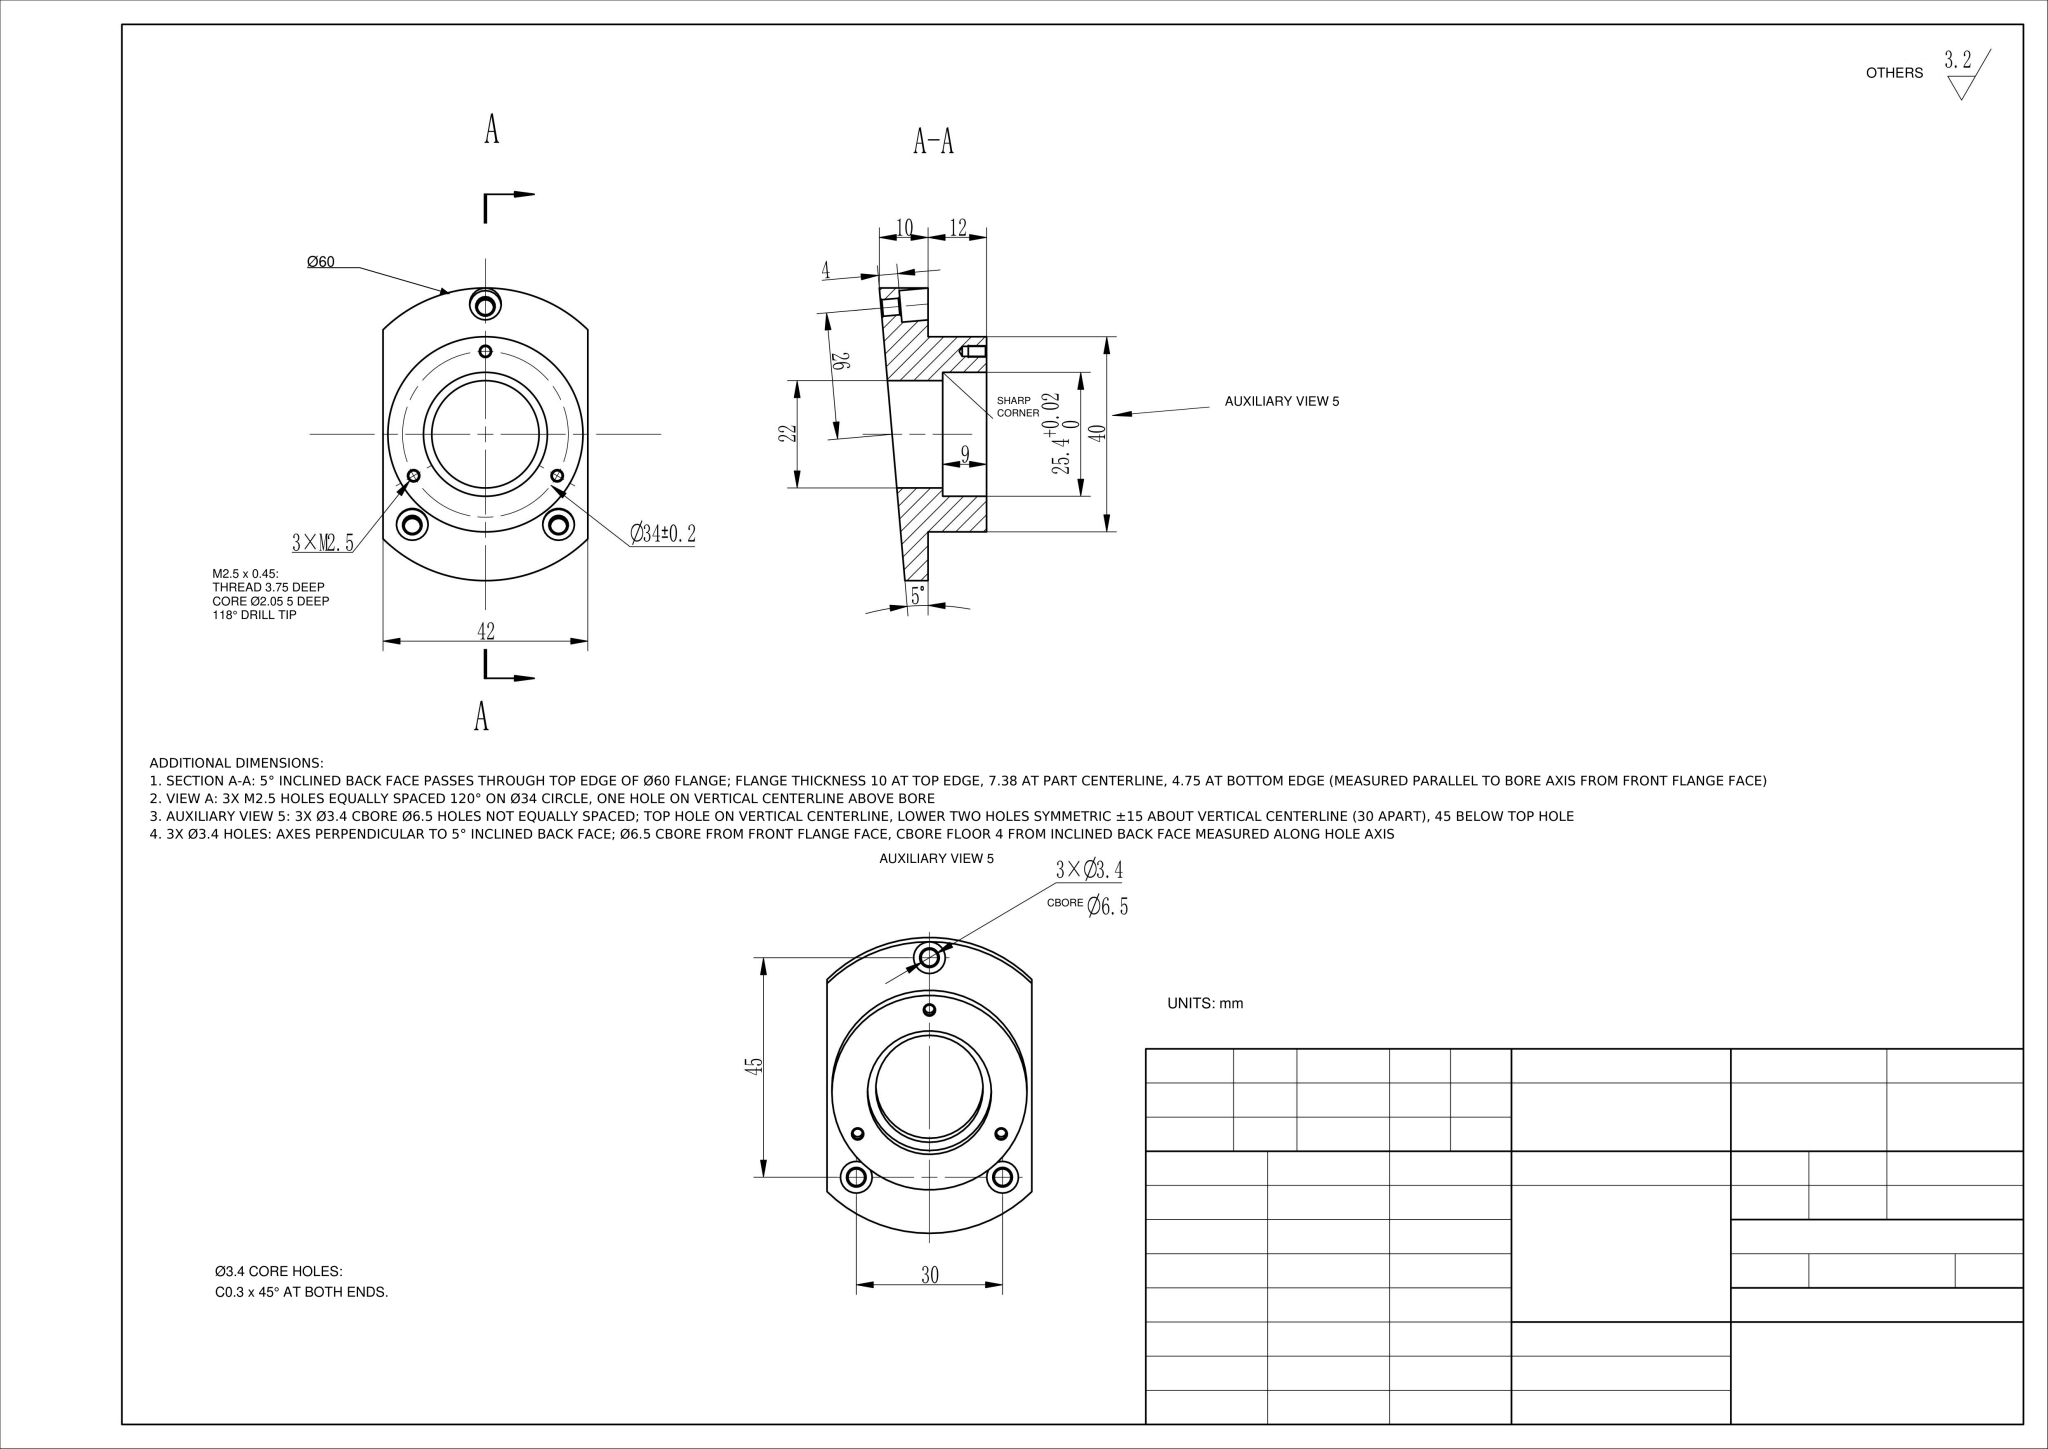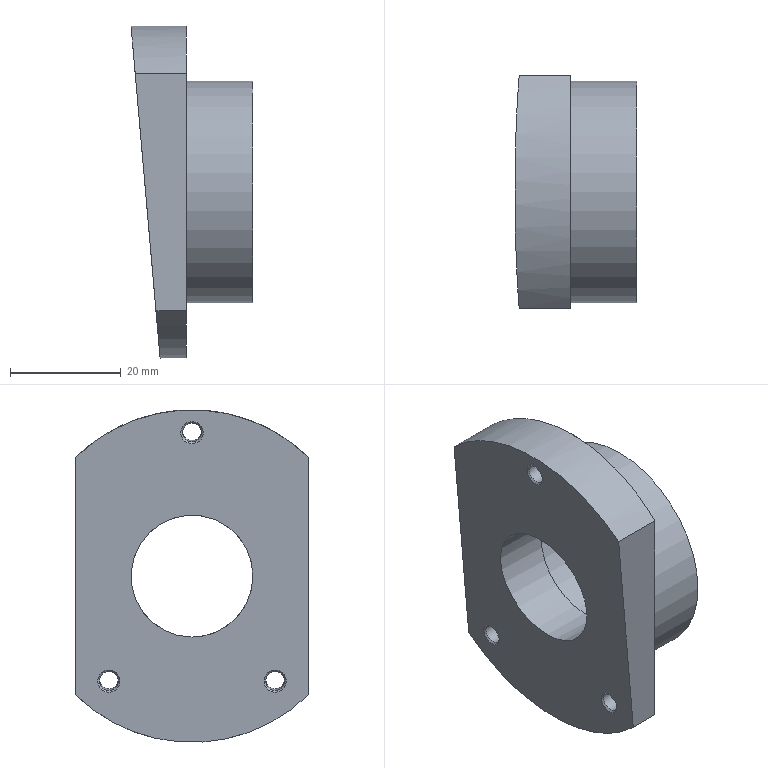Part | NX | mm | 1 solid | 35 faces | box 22 x 42 x 60 mm | volume 23038 mm3 | cylinder 14 | cone 12 | plane 9 | commonest cylinder face diameters 2.05 x3 6.5 x3 3.4 x3 60 x2 22 x1 40 x1 25.4 x1
STEP:
#1=CARTESIAN_POINT('',(0.,0.,0.));
#2=DIRECTION('',(0.,0.,1.));
#3=DIRECTION('',(1.,0.,0.));
#4=AXIS2_PLACEMENT_3D('',#1,#2,#3);
#5=(LENGTH_UNIT()NAMED_UNIT(*)SI_UNIT(.MILLI.,.METRE.));
#6=UNCERTAINTY_MEASURE_WITH_UNIT(LENGTH_MEASURE(0.00002),#5,'','');
#7=(NAMED_UNIT(*)PLANE_ANGLE_UNIT()SI_UNIT($,.RADIAN.));
#8=PLANE_ANGLE_MEASURE_WITH_UNIT(PLANE_ANGLE_MEASURE(0.01745),#7);
#9=DIMENSIONAL_EXPONENTS(0.,0.,0.,0.,0.,0.,0.);
#10=(CONVERSION_BASED_UNIT('',#8)NAMED_UNIT(#9)PLANE_ANGLE_UNIT());
#11=(NAMED_UNIT(*)SI_UNIT($,.STERADIAN.)SOLID_ANGLE_UNIT());
#12=(GEOMETRIC_REPRESENTATION_CONTEXT(3)GLOBAL_UNCERTAINTY_ASSIGNED_CONTEXT((#6))GLOBAL_UNIT_ASSIGNED_CONTEXT((#5,#10,#11))REPRESENTATION_CONTEXT('',''));
#13=SHAPE_REPRESENTATION('',(#4),#12);
#14=CARTESIAN_POINT('',(-5.501,-21.,-21.424));
#15=VERTEX_POINT('',#14);
#16=CARTESIAN_POINT('',(-9.25,-21.,21.424));
#17=VERTEX_POINT('',#16);
#18=CARTESIAN_POINT('',(-4.751,-21.,-30.));
#19=DIRECTION('',(-0.08716,0.,0.9962));
#20=VECTOR('',#19,1.);
#21=LINE('',#18,#20);
#22=EDGE_CURVE('',#15,#17,#21,.T.);
#23=ORIENTED_EDGE('',*,*,#22,.F.);
#24=CARTESIAN_POINT('',(0.,-21.,-21.424));
#25=VERTEX_POINT('',#24);
#26=CARTESIAN_POINT('',(-10.,-21.,-21.424));
#27=DIRECTION('',(1.,0.,0.));
#28=VECTOR('',#27,1.);
#29=LINE('',#26,#28);
#30=EDGE_CURVE('',#15,#25,#29,.T.);
#31=ORIENTED_EDGE('',*,*,#30,.T.);
#32=CARTESIAN_POINT('',(0.,-21.,21.424));
#33=VERTEX_POINT('',#32);
#34=CARTESIAN_POINT('',(0.,-21.,-21.424));
#35=DIRECTION('',(0.,-0.,1.));
#36=VECTOR('',#35,1.);
#37=LINE('',#34,#36);
#38=EDGE_CURVE('',#25,#33,#37,.T.);
#39=ORIENTED_EDGE('',*,*,#38,.T.);
#40=CARTESIAN_POINT('',(-10.,-21.,21.424));
#41=DIRECTION('',(1.,0.,0.));
#42=VECTOR('',#41,1.);
#43=LINE('',#40,#42);
#44=EDGE_CURVE('',#17,#33,#43,.T.);
#45=ORIENTED_EDGE('',*,*,#44,.F.);
#46=EDGE_LOOP('',(#23,#31,#39,#45));
#47=FACE_OUTER_BOUND('',#46,.T.);
#48=CARTESIAN_POINT('',(-10.,-21.,-21.424));
#49=DIRECTION('',(0.,1.,0.));
#50=DIRECTION('',(0.,-0.,1.));
#51=AXIS2_PLACEMENT_3D('',#48,#49,#50);
#52=PLANE('',#51);
#53=ADVANCED_FACE('',(#47),#52,.F.);
#54=CARTESIAN_POINT('',(3.,0.,-11.));
#55=VERTEX_POINT('',#54);
#56=CARTESIAN_POINT('',(3.,0.,0.));
#57=DIRECTION('',(-1.,0.,0.));
#58=DIRECTION('',(0.,0.,-1.));
#59=AXIS2_PLACEMENT_3D('',#56,#57,#58);
#60=CIRCLE('',#59,11.);
#61=EDGE_CURVE('',#55,#55,#60,.T.);
#62=ORIENTED_EDGE('',*,*,#61,.F.);
#63=EDGE_LOOP('',(#62));
#64=FACE_BOUND('',#63,.T.);
#65=CARTESIAN_POINT('',(-6.413,0.,-11.));
#66=VERTEX_POINT('',#65);
#67=CARTESIAN_POINT('',(-7.375,0.,0.));
#68=DIRECTION('',(0.9962,0.,0.08716));
#69=DIRECTION('',(0.08716,0.,-0.9962));
#70=AXIS2_PLACEMENT_3D('',#67,#68,#69);
#71=ELLIPSE('',#70,11.042,11.);
#72=EDGE_CURVE('',#66,#66,#71,.T.);
#73=ORIENTED_EDGE('',*,*,#72,.F.);
#74=EDGE_LOOP('',(#73));
#75=FACE_BOUND('',#74,.T.);
#76=CARTESIAN_POINT('',(-4.,0.,0.));
#77=DIRECTION('',(1.,0.,0.));
#78=DIRECTION('',(0.,0.,-1.));
#79=AXIS2_PLACEMENT_3D('',#76,#77,#78);
#80=CYLINDRICAL_SURFACE('',#79,11.);
#81=ADVANCED_FACE('',(#64,#75),#80,.F.);
#82=CARTESIAN_POINT('',(-9.25,21.,21.424));
#83=VERTEX_POINT('',#82);
#84=CARTESIAN_POINT('',(-7.375,0.,0.));
#85=DIRECTION('',(-0.9962,0.,-0.08716));
#86=DIRECTION('',(0.08716,0.,-0.9962));
#87=AXIS2_PLACEMENT_3D('',#84,#85,#86);
#88=ELLIPSE('',#87,30.115,30.);
#89=EDGE_CURVE('',#17,#83,#88,.T.);
#90=ORIENTED_EDGE('',*,*,#89,.F.);
#91=ORIENTED_EDGE('',*,*,#44,.T.);
#92=CARTESIAN_POINT('',(0.,21.,21.424));
#93=VERTEX_POINT('',#92);
#94=CARTESIAN_POINT('',(0.,0.,0.));
#95=DIRECTION('',(-1.,0.,0.));
#96=DIRECTION('',(0.,-1.,-0.));
#97=AXIS2_PLACEMENT_3D('',#94,#95,#96);
#98=CIRCLE('',#97,30.);
#99=EDGE_CURVE('',#33,#93,#98,.T.);
#100=ORIENTED_EDGE('',*,*,#99,.T.);
#101=CARTESIAN_POINT('',(-10.,21.,21.424));
#102=DIRECTION('',(1.,0.,0.));
#103=VECTOR('',#102,1.);
#104=LINE('',#101,#103);
#105=EDGE_CURVE('',#83,#93,#104,.T.);
#106=ORIENTED_EDGE('',*,*,#105,.F.);
#107=EDGE_LOOP('',(#90,#91,#100,#106));
#108=FACE_OUTER_BOUND('',#107,.T.);
#109=CARTESIAN_POINT('',(-10.,0.,0.));
#110=DIRECTION('',(1.,0.,0.));
#111=DIRECTION('',(0.,0.,-1.));
#112=AXIS2_PLACEMENT_3D('',#109,#110,#111);
#113=CYLINDRICAL_SURFACE('',#112,30.);
#114=ADVANCED_FACE('',(#108),#113,.T.);
#115=ORIENTED_EDGE('',*,*,#30,.F.);
#116=CARTESIAN_POINT('',(-5.501,21.,-21.424));
#117=VERTEX_POINT('',#116);
#118=CARTESIAN_POINT('',(-7.375,0.,0.));
#119=DIRECTION('',(-0.9962,0.,-0.08716));
#120=DIRECTION('',(0.08716,0.,-0.9962));
#121=AXIS2_PLACEMENT_3D('',#118,#119,#120);
#122=ELLIPSE('',#121,30.115,30.);
#123=EDGE_CURVE('',#117,#15,#122,.T.);
#124=ORIENTED_EDGE('',*,*,#123,.F.);
#125=CARTESIAN_POINT('',(0.,21.,-21.424));
#126=VERTEX_POINT('',#125);
#127=CARTESIAN_POINT('',(-10.,21.,-21.424));
#128=DIRECTION('',(1.,0.,0.));
#129=VECTOR('',#128,1.);
#130=LINE('',#127,#129);
#131=EDGE_CURVE('',#117,#126,#130,.T.);
#132=ORIENTED_EDGE('',*,*,#131,.T.);
#133=CARTESIAN_POINT('',(0.,0.,0.));
#134=DIRECTION('',(-1.,0.,0.));
#135=DIRECTION('',(0.,-1.,-0.));
#136=AXIS2_PLACEMENT_3D('',#133,#134,#135);
#137=CIRCLE('',#136,30.);
#138=EDGE_CURVE('',#126,#25,#137,.T.);
#139=ORIENTED_EDGE('',*,*,#138,.T.);
#140=EDGE_LOOP('',(#115,#124,#132,#139));
#141=FACE_OUTER_BOUND('',#140,.T.);
#142=CARTESIAN_POINT('',(-10.,0.,0.));
#143=DIRECTION('',(1.,0.,0.));
#144=DIRECTION('',(0.,0.,-1.));
#145=AXIS2_PLACEMENT_3D('',#142,#143,#144);
#146=CYLINDRICAL_SURFACE('',#145,30.);
#147=ADVANCED_FACE('',(#141),#146,.T.);
#148=CARTESIAN_POINT('',(12.,20.,-0.));
#149=VERTEX_POINT('',#148);
#150=CARTESIAN_POINT('',(12.,0.,0.));
#151=DIRECTION('',(1.,0.,0.));
#152=DIRECTION('',(0.,1.,-0.));
#153=AXIS2_PLACEMENT_3D('',#150,#151,#152);
#154=CIRCLE('',#153,20.);
#155=EDGE_CURVE('',#149,#149,#154,.T.);
#156=ORIENTED_EDGE('',*,*,#155,.F.);
#157=EDGE_LOOP('',(#156));
#158=FACE_BOUND('',#157,.T.);
#159=CARTESIAN_POINT('',(0.,20.,-0.));
#160=VERTEX_POINT('',#159);
#161=CARTESIAN_POINT('',(0.,0.,0.));
#162=DIRECTION('',(1.,0.,0.));
#163=DIRECTION('',(0.,1.,-0.));
#164=AXIS2_PLACEMENT_3D('',#161,#162,#163);
#165=CIRCLE('',#164,20.);
#166=EDGE_CURVE('',#160,#160,#165,.T.);
#167=ORIENTED_EDGE('',*,*,#166,.T.);
#168=EDGE_LOOP('',(#167));
#169=FACE_BOUND('',#168,.T.);
#170=CARTESIAN_POINT('',(12.,0.,0.));
#171=DIRECTION('',(-1.,0.,0.));
#172=DIRECTION('',(0.,0.,1.));
#173=AXIS2_PLACEMENT_3D('',#170,#171,#172);
#174=CYLINDRICAL_SURFACE('',#173,20.);
#175=ADVANCED_FACE('',(#158,#169),#174,.T.);
#176=CARTESIAN_POINT('',(12.,14.722,-9.75));
#177=VERTEX_POINT('',#176);
#178=CARTESIAN_POINT('',(12.,14.722,-8.5));
#179=DIRECTION('',(-1.,0.,0.));
#180=DIRECTION('',(0.,0.,-1.));
#181=AXIS2_PLACEMENT_3D('',#178,#179,#180);
#182=CIRCLE('',#181,1.25);
#183=EDGE_CURVE('',#177,#177,#182,.T.);
#184=ORIENTED_EDGE('',*,*,#183,.T.);
#185=EDGE_LOOP('',(#184));
#186=FACE_BOUND('',#185,.T.);
#187=CARTESIAN_POINT('',(12.,0.,15.75));
#188=VERTEX_POINT('',#187);
#189=CARTESIAN_POINT('',(12.,0.,17.));
#190=DIRECTION('',(-1.,0.,0.));
#191=DIRECTION('',(0.,0.,-1.));
#192=AXIS2_PLACEMENT_3D('',#189,#190,#191);
#193=CIRCLE('',#192,1.25);
#194=EDGE_CURVE('',#188,#188,#193,.T.);
#195=ORIENTED_EDGE('',*,*,#194,.T.);
#196=EDGE_LOOP('',(#195));
#197=FACE_BOUND('',#196,.T.);
#198=CARTESIAN_POINT('',(12.,-14.722,-9.75));
#199=VERTEX_POINT('',#198);
#200=CARTESIAN_POINT('',(12.,-14.722,-8.5));
#201=DIRECTION('',(-1.,0.,0.));
#202=DIRECTION('',(0.,0.,-1.));
#203=AXIS2_PLACEMENT_3D('',#200,#201,#202);
#204=CIRCLE('',#203,1.25);
#205=EDGE_CURVE('',#199,#199,#204,.T.);
#206=ORIENTED_EDGE('',*,*,#205,.T.);
#207=EDGE_LOOP('',(#206));
#208=FACE_BOUND('',#207,.T.);
#209=CARTESIAN_POINT('',(12.,12.7,-0.));
#210=VERTEX_POINT('',#209);
#211=CARTESIAN_POINT('',(12.,0.,0.));
#212=DIRECTION('',(1.,0.,0.));
#213=DIRECTION('',(0.,1.,-0.));
#214=AXIS2_PLACEMENT_3D('',#211,#212,#213);
#215=CIRCLE('',#214,12.7);
#216=EDGE_CURVE('',#210,#210,#215,.T.);
#217=ORIENTED_EDGE('',*,*,#216,.F.);
#218=EDGE_LOOP('',(#217));
#219=FACE_BOUND('',#218,.T.);
#220=ORIENTED_EDGE('',*,*,#155,.T.);
#221=EDGE_LOOP('',(#220));
#222=FACE_BOUND('',#221,.T.);
#223=CARTESIAN_POINT('',(12.,0.,0.));
#224=DIRECTION('',(1.,0.,0.));
#225=DIRECTION('',(0.,0.,-1.));
#226=AXIS2_PLACEMENT_3D('',#223,#224,#225);
#227=PLANE('',#226);
#228=ADVANCED_FACE('',(#186,#197,#208,#219,#222),#227,.T.);
#229=CARTESIAN_POINT('',(3.,12.7,-0.));
#230=VERTEX_POINT('',#229);
#231=CARTESIAN_POINT('',(3.,0.,0.));
#232=DIRECTION('',(-1.,0.,0.));
#233=DIRECTION('',(0.,1.,-0.));
#234=AXIS2_PLACEMENT_3D('',#231,#232,#233);
#235=CIRCLE('',#234,12.7);
#236=EDGE_CURVE('',#230,#230,#235,.T.);
#237=ORIENTED_EDGE('',*,*,#236,.F.);
#238=EDGE_LOOP('',(#237));
#239=FACE_BOUND('',#238,.T.);
#240=ORIENTED_EDGE('',*,*,#61,.T.);
#241=EDGE_LOOP('',(#240));
#242=FACE_BOUND('',#241,.T.);
#243=CARTESIAN_POINT('',(3.,0.,0.));
#244=DIRECTION('',(1.,0.,0.));
#245=DIRECTION('',(0.,0.,-1.));
#246=AXIS2_PLACEMENT_3D('',#243,#244,#245);
#247=PLANE('',#246);
#248=ADVANCED_FACE('',(#239,#242),#247,.T.);
#249=ORIENTED_EDGE('',*,*,#236,.T.);
#250=EDGE_LOOP('',(#249));
#251=FACE_BOUND('',#250,.T.);
#252=ORIENTED_EDGE('',*,*,#216,.T.);
#253=EDGE_LOOP('',(#252));
#254=FACE_BOUND('',#253,.T.);
#255=CARTESIAN_POINT('',(3.,0.,0.));
#256=DIRECTION('',(1.,0.,0.));
#257=DIRECTION('',(0.,0.,-1.));
#258=AXIS2_PLACEMENT_3D('',#255,#256,#257);
#259=CYLINDRICAL_SURFACE('',#258,12.7);
#260=ADVANCED_FACE('',(#251,#254),#259,.F.);
#261=ORIENTED_EDGE('',*,*,#131,.F.);
#262=CARTESIAN_POINT('',(-4.751,21.,-30.));
#263=DIRECTION('',(-0.08716,0.,0.9962));
#264=VECTOR('',#263,1.);
#265=LINE('',#262,#264);
#266=EDGE_CURVE('',#117,#83,#265,.T.);
#267=ORIENTED_EDGE('',*,*,#266,.T.);
#268=ORIENTED_EDGE('',*,*,#105,.T.);
#269=CARTESIAN_POINT('',(0.,21.,21.424));
#270=DIRECTION('',(0.,0.,-1.));
#271=VECTOR('',#270,1.);
#272=LINE('',#269,#271);
#273=EDGE_CURVE('',#93,#126,#272,.T.);
#274=ORIENTED_EDGE('',*,*,#273,.T.);
#275=EDGE_LOOP('',(#261,#267,#268,#274));
#276=FACE_OUTER_BOUND('',#275,.T.);
#277=CARTESIAN_POINT('',(-10.,21.,21.424));
#278=DIRECTION('',(0.,-1.,-0.));
#279=DIRECTION('',(0.,0.,-1.));
#280=AXIS2_PLACEMENT_3D('',#277,#278,#279);
#281=PLANE('',#280);
#282=ADVANCED_FACE('',(#276),#281,.F.);
#283=CARTESIAN_POINT('',(0.,15.,-21.72));
#284=VERTEX_POINT('',#283);
#285=CARTESIAN_POINT('',(0.,15.,-18.458));
#286=DIRECTION('',(-1.,0.,0.));
#287=DIRECTION('',(0.,0.,-1.));
#288=AXIS2_PLACEMENT_3D('',#285,#286,#287);
#289=ELLIPSE('',#288,3.262,3.25);
#290=EDGE_CURVE('',#284,#284,#289,.T.);
#291=ORIENTED_EDGE('',*,*,#290,.T.);
#292=EDGE_LOOP('',(#291));
#293=FACE_BOUND('',#292,.T.);
#294=CARTESIAN_POINT('',(0.,0.,23.452));
#295=VERTEX_POINT('',#294);
#296=CARTESIAN_POINT('',(0.,0.,26.714));
#297=DIRECTION('',(-1.,0.,0.));
#298=DIRECTION('',(0.,0.,-1.));
#299=AXIS2_PLACEMENT_3D('',#296,#297,#298);
#300=ELLIPSE('',#299,3.262,3.25);
#301=EDGE_CURVE('',#295,#295,#300,.T.);
#302=ORIENTED_EDGE('',*,*,#301,.T.);
#303=EDGE_LOOP('',(#302));
#304=FACE_BOUND('',#303,.T.);
#305=CARTESIAN_POINT('',(0.,-15.,-21.72));
#306=VERTEX_POINT('',#305);
#307=CARTESIAN_POINT('',(0.,-15.,-18.458));
#308=DIRECTION('',(-1.,0.,0.));
#309=DIRECTION('',(0.,0.,-1.));
#310=AXIS2_PLACEMENT_3D('',#307,#308,#309);
#311=ELLIPSE('',#310,3.262,3.25);
#312=EDGE_CURVE('',#306,#306,#311,.T.);
#313=ORIENTED_EDGE('',*,*,#312,.T.);
#314=EDGE_LOOP('',(#313));
#315=FACE_BOUND('',#314,.T.);
#316=ORIENTED_EDGE('',*,*,#166,.F.);
#317=EDGE_LOOP('',(#316));
#318=FACE_BOUND('',#317,.T.);
#319=ORIENTED_EDGE('',*,*,#99,.F.);
#320=ORIENTED_EDGE('',*,*,#38,.F.);
#321=ORIENTED_EDGE('',*,*,#138,.F.);
#322=ORIENTED_EDGE('',*,*,#273,.F.);
#323=EDGE_LOOP('',(#319,#320,#321,#322));
#324=FACE_BOUND('',#323,.T.);
#325=CARTESIAN_POINT('',(0.,0.,0.));
#326=DIRECTION('',(-1.,0.,0.));
#327=DIRECTION('',(0.,0.,1.));
#328=AXIS2_PLACEMENT_3D('',#325,#326,#327);
#329=PLANE('',#328);
#330=ADVANCED_FACE('',(#293,#304,#315,#318,#324),#329,.F.);
#331=CARTESIAN_POINT('',(-5.891,15.,-16.966));
#332=VERTEX_POINT('',#331);
#333=CARTESIAN_POINT('',(-5.717,15.,-18.958));
#334=DIRECTION('',(0.9962,0.,0.08716));
#335=DIRECTION('',(-0.08716,0.,0.9962));
#336=AXIS2_PLACEMENT_3D('',#333,#334,#335);
#337=CIRCLE('',#336,2.);
#338=EDGE_CURVE('',#332,#332,#337,.T.);
#339=ORIENTED_EDGE('',*,*,#338,.T.);
#340=EDGE_LOOP('',(#339));
#341=FACE_BOUND('',#340,.T.);
#342=CARTESIAN_POINT('',(-5.891,-15.,-16.966));
#343=VERTEX_POINT('',#342);
#344=CARTESIAN_POINT('',(-5.717,-15.,-18.958));
#345=DIRECTION('',(0.9962,0.,0.08716));
#346=DIRECTION('',(-0.08716,0.,0.9962));
#347=AXIS2_PLACEMENT_3D('',#344,#345,#346);
#348=CIRCLE('',#347,2.);
#349=EDGE_CURVE('',#343,#343,#348,.T.);
#350=ORIENTED_EDGE('',*,*,#349,.T.);
#351=EDGE_LOOP('',(#350));
#352=FACE_BOUND('',#351,.T.);
#353=CARTESIAN_POINT('',(-9.813,0.,27.863));
#354=VERTEX_POINT('',#353);
#355=CARTESIAN_POINT('',(-9.639,0.,25.871));
#356=DIRECTION('',(0.9962,0.,0.08716));
#357=DIRECTION('',(-0.08716,0.,0.9962));
#358=AXIS2_PLACEMENT_3D('',#355,#356,#357);
#359=CIRCLE('',#358,2.);
#360=EDGE_CURVE('',#354,#354,#359,.T.);
#361=ORIENTED_EDGE('',*,*,#360,.T.);
#362=EDGE_LOOP('',(#361));
#363=FACE_BOUND('',#362,.T.);
#364=ORIENTED_EDGE('',*,*,#89,.T.);
#365=ORIENTED_EDGE('',*,*,#266,.F.);
#366=ORIENTED_EDGE('',*,*,#123,.T.);
#367=ORIENTED_EDGE('',*,*,#22,.T.);
#368=EDGE_LOOP('',(#364,#365,#366,#367));
#369=FACE_BOUND('',#368,.T.);
#370=ORIENTED_EDGE('',*,*,#72,.T.);
#371=EDGE_LOOP('',(#370));
#372=FACE_BOUND('',#371,.T.);
#373=CARTESIAN_POINT('',(-4.751,-21.,-30.));
#374=DIRECTION('',(-0.9962,0.,-0.08716));
#375=DIRECTION('',(-0.08716,0.,0.9962));
#376=AXIS2_PLACEMENT_3D('',#373,#374,#375);
#377=PLANE('',#376);
#378=ADVANCED_FACE('',(#341,#352,#363,#369,#372),#377,.T.);
#379=CARTESIAN_POINT('',(7.,-14.722,-7.475));
#380=VERTEX_POINT('',#379);
#381=CARTESIAN_POINT('',(7.,-14.722,-8.5));
#382=DIRECTION('',(1.,0.,0.));
#383=DIRECTION('',(0.,0.,1.));
#384=AXIS2_PLACEMENT_3D('',#381,#382,#383);
#385=CIRCLE('',#384,1.025);
#386=EDGE_CURVE('',#380,#380,#385,.T.);
#387=ORIENTED_EDGE('',*,*,#386,.T.);
#388=EDGE_LOOP('',(#387));
#389=FACE_BOUND('',#388,.T.);
#390=CARTESIAN_POINT('',(6.384,-14.722,-8.5));
#391=VERTEX_POINT('',#390);
#392=VERTEX_LOOP('',#391);
#393=FACE_BOUND('',#392,.T.);
#394=CARTESIAN_POINT('',(7.,-14.722,-8.5));
#395=DIRECTION('',(1.,0.,0.));
#396=DIRECTION('',(-0.,0.,-1.));
#397=AXIS2_PLACEMENT_3D('',#394,#395,#396);
#398=CONICAL_SURFACE('',#397,1.025,59.);
#399=ADVANCED_FACE('',(#389,#393),#398,.F.);
#400=CARTESIAN_POINT('',(11.775,-14.722,-9.525));
#401=VERTEX_POINT('',#400);
#402=CARTESIAN_POINT('',(11.775,-14.722,-8.5));
#403=DIRECTION('',(1.,0.,0.));
#404=DIRECTION('',(0.,0.,-1.));
#405=AXIS2_PLACEMENT_3D('',#402,#403,#404);
#406=CIRCLE('',#405,1.025);
#407=EDGE_CURVE('',#401,#401,#406,.T.);
#408=ORIENTED_EDGE('',*,*,#407,.T.);
#409=EDGE_LOOP('',(#408));
#410=FACE_BOUND('',#409,.T.);
#411=ORIENTED_EDGE('',*,*,#386,.F.);
#412=EDGE_LOOP('',(#411));
#413=FACE_BOUND('',#412,.T.);
#414=CARTESIAN_POINT('',(12.,-14.722,-8.5));
#415=DIRECTION('',(-1.,0.,0.));
#416=DIRECTION('',(0.,0.,1.));
#417=AXIS2_PLACEMENT_3D('',#414,#415,#416);
#418=CYLINDRICAL_SURFACE('',#417,1.025);
#419=ADVANCED_FACE('',(#410,#413),#418,.F.);
#420=ORIENTED_EDGE('',*,*,#407,.F.);
#421=EDGE_LOOP('',(#420));
#422=FACE_BOUND('',#421,.T.);
#423=ORIENTED_EDGE('',*,*,#205,.F.);
#424=EDGE_LOOP('',(#423));
#425=FACE_BOUND('',#424,.T.);
#426=CARTESIAN_POINT('',(12.,-14.722,-8.5));
#427=DIRECTION('',(1.,0.,0.));
#428=DIRECTION('',(0.,0.,-1.));
#429=AXIS2_PLACEMENT_3D('',#426,#427,#428);
#430=CONICAL_SURFACE('',#429,1.25,45.);
#431=ADVANCED_FACE('',(#422,#425),#430,.F.);
#432=CARTESIAN_POINT('',(7.,0.,18.025));
#433=VERTEX_POINT('',#432);
#434=CARTESIAN_POINT('',(7.,0.,17.));
#435=DIRECTION('',(1.,0.,0.));
#436=DIRECTION('',(0.,0.,1.));
#437=AXIS2_PLACEMENT_3D('',#434,#435,#436);
#438=CIRCLE('',#437,1.025);
#439=EDGE_CURVE('',#433,#433,#438,.T.);
#440=ORIENTED_EDGE('',*,*,#439,.T.);
#441=EDGE_LOOP('',(#440));
#442=FACE_BOUND('',#441,.T.);
#443=CARTESIAN_POINT('',(6.384,0.,17.));
#444=VERTEX_POINT('',#443);
#445=VERTEX_LOOP('',#444);
#446=FACE_BOUND('',#445,.T.);
#447=CARTESIAN_POINT('',(7.,0.,17.));
#448=DIRECTION('',(1.,0.,0.));
#449=DIRECTION('',(-0.,0.,-1.));
#450=AXIS2_PLACEMENT_3D('',#447,#448,#449);
#451=CONICAL_SURFACE('',#450,1.025,59.);
#452=ADVANCED_FACE('',(#442,#446),#451,.F.);
#453=CARTESIAN_POINT('',(11.775,0.,15.975));
#454=VERTEX_POINT('',#453);
#455=CARTESIAN_POINT('',(11.775,0.,17.));
#456=DIRECTION('',(1.,0.,0.));
#457=DIRECTION('',(0.,0.,-1.));
#458=AXIS2_PLACEMENT_3D('',#455,#456,#457);
#459=CIRCLE('',#458,1.025);
#460=EDGE_CURVE('',#454,#454,#459,.T.);
#461=ORIENTED_EDGE('',*,*,#460,.T.);
#462=EDGE_LOOP('',(#461));
#463=FACE_BOUND('',#462,.T.);
#464=ORIENTED_EDGE('',*,*,#439,.F.);
#465=EDGE_LOOP('',(#464));
#466=FACE_BOUND('',#465,.T.);
#467=CARTESIAN_POINT('',(12.,0.,17.));
#468=DIRECTION('',(-1.,0.,0.));
#469=DIRECTION('',(0.,0.,1.));
#470=AXIS2_PLACEMENT_3D('',#467,#468,#469);
#471=CYLINDRICAL_SURFACE('',#470,1.025);
#472=ADVANCED_FACE('',(#463,#466),#471,.F.);
#473=ORIENTED_EDGE('',*,*,#460,.F.);
#474=EDGE_LOOP('',(#473));
#475=FACE_BOUND('',#474,.T.);
#476=ORIENTED_EDGE('',*,*,#194,.F.);
#477=EDGE_LOOP('',(#476));
#478=FACE_BOUND('',#477,.T.);
#479=CARTESIAN_POINT('',(12.,0.,17.));
#480=DIRECTION('',(1.,0.,0.));
#481=DIRECTION('',(0.,0.,-1.));
#482=AXIS2_PLACEMENT_3D('',#479,#480,#481);
#483=CONICAL_SURFACE('',#482,1.25,45.);
#484=ADVANCED_FACE('',(#475,#478),#483,.F.);
#485=CARTESIAN_POINT('',(7.,14.722,-7.475));
#486=VERTEX_POINT('',#485);
#487=CARTESIAN_POINT('',(7.,14.722,-8.5));
#488=DIRECTION('',(1.,0.,0.));
#489=DIRECTION('',(0.,0.,1.));
#490=AXIS2_PLACEMENT_3D('',#487,#488,#489);
#491=CIRCLE('',#490,1.025);
#492=EDGE_CURVE('',#486,#486,#491,.T.);
#493=ORIENTED_EDGE('',*,*,#492,.T.);
#494=EDGE_LOOP('',(#493));
#495=FACE_BOUND('',#494,.T.);
#496=CARTESIAN_POINT('',(6.384,14.722,-8.5));
#497=VERTEX_POINT('',#496);
#498=VERTEX_LOOP('',#497);
#499=FACE_BOUND('',#498,.T.);
#500=CARTESIAN_POINT('',(7.,14.722,-8.5));
#501=DIRECTION('',(1.,0.,0.));
#502=DIRECTION('',(-0.,0.,-1.));
#503=AXIS2_PLACEMENT_3D('',#500,#501,#502);
#504=CONICAL_SURFACE('',#503,1.025,59.);
#505=ADVANCED_FACE('',(#495,#499),#504,.F.);
#506=CARTESIAN_POINT('',(11.775,14.722,-9.525));
#507=VERTEX_POINT('',#506);
#508=CARTESIAN_POINT('',(11.775,14.722,-8.5));
#509=DIRECTION('',(1.,0.,0.));
#510=DIRECTION('',(0.,0.,-1.));
#511=AXIS2_PLACEMENT_3D('',#508,#509,#510);
#512=CIRCLE('',#511,1.025);
#513=EDGE_CURVE('',#507,#507,#512,.T.);
#514=ORIENTED_EDGE('',*,*,#513,.T.);
#515=EDGE_LOOP('',(#514));
#516=FACE_BOUND('',#515,.T.);
#517=ORIENTED_EDGE('',*,*,#492,.F.);
#518=EDGE_LOOP('',(#517));
#519=FACE_BOUND('',#518,.T.);
#520=CARTESIAN_POINT('',(12.,14.722,-8.5));
#521=DIRECTION('',(-1.,0.,0.));
#522=DIRECTION('',(0.,0.,1.));
#523=AXIS2_PLACEMENT_3D('',#520,#521,#522);
#524=CYLINDRICAL_SURFACE('',#523,1.025);
#525=ADVANCED_FACE('',(#516,#519),#524,.F.);
#526=ORIENTED_EDGE('',*,*,#513,.F.);
#527=EDGE_LOOP('',(#526));
#528=FACE_BOUND('',#527,.T.);
#529=ORIENTED_EDGE('',*,*,#183,.F.);
#530=EDGE_LOOP('',(#529));
#531=FACE_BOUND('',#530,.T.);
#532=CARTESIAN_POINT('',(12.,14.722,-8.5));
#533=DIRECTION('',(1.,0.,0.));
#534=DIRECTION('',(0.,0.,-1.));
#535=AXIS2_PLACEMENT_3D('',#532,#533,#534);
#536=CONICAL_SURFACE('',#535,1.25,45.);
#537=ADVANCED_FACE('',(#528,#531),#536,.F.);
#538=CARTESIAN_POINT('',(-2.015,-15.,-15.372));
#539=VERTEX_POINT('',#538);
#540=CARTESIAN_POINT('',(-1.732,-15.,-18.609));
#541=DIRECTION('',(0.9962,0.,0.08716));
#542=DIRECTION('',(-0.08716,0.,0.9962));
#543=AXIS2_PLACEMENT_3D('',#540,#541,#542);
#544=CIRCLE('',#543,3.25);
#545=EDGE_CURVE('',#539,#539,#544,.T.);
#546=ORIENTED_EDGE('',*,*,#545,.F.);
#547=EDGE_LOOP('',(#546));
#548=FACE_BOUND('',#547,.T.);
#549=ORIENTED_EDGE('',*,*,#312,.F.);
#550=EDGE_LOOP('',(#549));
#551=FACE_BOUND('',#550,.T.);
#552=CARTESIAN_POINT('',(4.245,-15.,-18.086));
#553=DIRECTION('',(-0.9962,0.,-0.08716));
#554=DIRECTION('',(-0.08716,0.,0.9962));
#555=AXIS2_PLACEMENT_3D('',#552,#553,#554);
#556=CYLINDRICAL_SURFACE('',#555,3.25);
#557=ADVANCED_FACE('',(#548,#551),#556,.F.);
#558=CARTESIAN_POINT('',(-1.906,-15.,-16.617));
#559=VERTEX_POINT('',#558);
#560=CARTESIAN_POINT('',(-1.732,-15.,-18.609));
#561=DIRECTION('',(-0.9962,0.,-0.08716));
#562=DIRECTION('',(-0.08716,0.,0.9962));
#563=AXIS2_PLACEMENT_3D('',#560,#561,#562);
#564=CIRCLE('',#563,2.);
#565=EDGE_CURVE('',#559,#559,#564,.T.);
#566=ORIENTED_EDGE('',*,*,#565,.T.);
#567=EDGE_LOOP('',(#566));
#568=FACE_BOUND('',#567,.T.);
#569=ORIENTED_EDGE('',*,*,#545,.T.);
#570=EDGE_LOOP('',(#569));
#571=FACE_BOUND('',#570,.T.);
#572=CARTESIAN_POINT('',(-1.732,-15.,-18.609));
#573=DIRECTION('',(-0.9962,0.,-0.08716));
#574=DIRECTION('',(-0.08716,0.,0.9962));
#575=AXIS2_PLACEMENT_3D('',#572,#573,#574);
#576=PLANE('',#575);
#577=ADVANCED_FACE('',(#568,#571),#576,.F.);
#578=CARTESIAN_POINT('',(-5.937,0.,29.457));
#579=VERTEX_POINT('',#578);
#580=CARTESIAN_POINT('',(-5.654,0.,26.219));
#581=DIRECTION('',(0.9962,0.,0.08716));
#582=DIRECTION('',(-0.08716,0.,0.9962));
#583=AXIS2_PLACEMENT_3D('',#580,#581,#582);
#584=CIRCLE('',#583,3.25);
#585=EDGE_CURVE('',#579,#579,#584,.T.);
#586=ORIENTED_EDGE('',*,*,#585,.F.);
#587=EDGE_LOOP('',(#586));
#588=FACE_BOUND('',#587,.T.);
#589=ORIENTED_EDGE('',*,*,#301,.F.);
#590=EDGE_LOOP('',(#589));
#591=FACE_BOUND('',#590,.T.);
#592=CARTESIAN_POINT('',(0.3232,0.,26.742));
#593=DIRECTION('',(-0.9962,0.,-0.08716));
#594=DIRECTION('',(-0.08716,0.,0.9962));
#595=AXIS2_PLACEMENT_3D('',#592,#593,#594);
#596=CYLINDRICAL_SURFACE('',#595,3.25);
#597=ADVANCED_FACE('',(#588,#591),#596,.F.);
#598=CARTESIAN_POINT('',(-5.828,0.,28.212));
#599=VERTEX_POINT('',#598);
#600=CARTESIAN_POINT('',(-5.654,0.,26.219));
#601=DIRECTION('',(-0.9962,0.,-0.08716));
#602=DIRECTION('',(-0.08716,0.,0.9962));
#603=AXIS2_PLACEMENT_3D('',#600,#601,#602);
#604=CIRCLE('',#603,2.);
#605=EDGE_CURVE('',#599,#599,#604,.T.);
#606=ORIENTED_EDGE('',*,*,#605,.T.);
#607=EDGE_LOOP('',(#606));
#608=FACE_BOUND('',#607,.T.);
#609=ORIENTED_EDGE('',*,*,#585,.T.);
#610=EDGE_LOOP('',(#609));
#611=FACE_BOUND('',#610,.T.);
#612=CARTESIAN_POINT('',(-5.654,0.,26.219));
#613=DIRECTION('',(-0.9962,0.,-0.08716));
#614=DIRECTION('',(-0.08716,0.,0.9962));
#615=AXIS2_PLACEMENT_3D('',#612,#613,#614);
#616=PLANE('',#615);
#617=ADVANCED_FACE('',(#608,#611),#616,.F.);
#618=CARTESIAN_POINT('',(-2.015,15.,-15.372));
#619=VERTEX_POINT('',#618);
#620=CARTESIAN_POINT('',(-1.732,15.,-18.609));
#621=DIRECTION('',(0.9962,0.,0.08716));
#622=DIRECTION('',(-0.08716,0.,0.9962));
#623=AXIS2_PLACEMENT_3D('',#620,#621,#622);
#624=CIRCLE('',#623,3.25);
#625=EDGE_CURVE('',#619,#619,#624,.T.);
#626=ORIENTED_EDGE('',*,*,#625,.F.);
#627=EDGE_LOOP('',(#626));
#628=FACE_BOUND('',#627,.T.);
#629=ORIENTED_EDGE('',*,*,#290,.F.);
#630=EDGE_LOOP('',(#629));
#631=FACE_BOUND('',#630,.T.);
#632=CARTESIAN_POINT('',(4.245,15.,-18.086));
#633=DIRECTION('',(-0.9962,0.,-0.08716));
#634=DIRECTION('',(-0.08716,0.,0.9962));
#635=AXIS2_PLACEMENT_3D('',#632,#633,#634);
#636=CYLINDRICAL_SURFACE('',#635,3.25);
#637=ADVANCED_FACE('',(#628,#631),#636,.F.);
#638=CARTESIAN_POINT('',(-1.906,15.,-16.617));
#639=VERTEX_POINT('',#638);
#640=CARTESIAN_POINT('',(-1.732,15.,-18.609));
#641=DIRECTION('',(-0.9962,0.,-0.08716));
#642=DIRECTION('',(-0.08716,0.,0.9962));
#643=AXIS2_PLACEMENT_3D('',#640,#641,#642);
#644=CIRCLE('',#643,2.);
#645=EDGE_CURVE('',#639,#639,#644,.T.);
#646=ORIENTED_EDGE('',*,*,#645,.T.);
#647=EDGE_LOOP('',(#646));
#648=FACE_BOUND('',#647,.T.);
#649=ORIENTED_EDGE('',*,*,#625,.T.);
#650=EDGE_LOOP('',(#649));
#651=FACE_BOUND('',#650,.T.);
#652=CARTESIAN_POINT('',(-1.732,15.,-18.609));
#653=DIRECTION('',(-0.9962,0.,-0.08716));
#654=DIRECTION('',(-0.08716,0.,0.9962));
#655=AXIS2_PLACEMENT_3D('',#652,#653,#654);
#656=PLANE('',#655);
#657=ADVANCED_FACE('',(#648,#651),#656,.F.);
#658=CARTESIAN_POINT('',(-9.488,0.,27.59));
#659=VERTEX_POINT('',#658);
#660=CARTESIAN_POINT('',(-9.34,0.,25.897));
#661=DIRECTION('',(-0.9962,0.,-0.08716));
#662=DIRECTION('',(-0.08716,0.,0.9962));
#663=AXIS2_PLACEMENT_3D('',#660,#661,#662);
#664=CIRCLE('',#663,1.7);
#665=EDGE_CURVE('',#659,#659,#664,.T.);
#666=ORIENTED_EDGE('',*,*,#665,.T.);
#667=EDGE_LOOP('',(#666));
#668=FACE_BOUND('',#667,.T.);
#669=CARTESIAN_POINT('',(-6.101,0.,27.887));
#670=VERTEX_POINT('',#669);
#671=CARTESIAN_POINT('',(-5.953,0.,26.193));
#672=DIRECTION('',(0.9962,0.,0.08716));
#673=DIRECTION('',(-0.08716,0.,0.9962));
#674=AXIS2_PLACEMENT_3D('',#671,#672,#673);
#675=CIRCLE('',#674,1.7);
#676=EDGE_CURVE('',#670,#670,#675,.T.);
#677=ORIENTED_EDGE('',*,*,#676,.T.);
#678=EDGE_LOOP('',(#677));
#679=FACE_BOUND('',#678,.T.);
#680=CARTESIAN_POINT('',(-5.654,0.,26.219));
#681=DIRECTION('',(-0.9962,0.,-0.08716));
#682=DIRECTION('',(-0.08716,0.,0.9962));
#683=AXIS2_PLACEMENT_3D('',#680,#681,#682);
#684=CYLINDRICAL_SURFACE('',#683,1.7);
#685=ADVANCED_FACE('',(#668,#679),#684,.F.);
#686=ORIENTED_EDGE('',*,*,#676,.F.);
#687=EDGE_LOOP('',(#686));
#688=FACE_BOUND('',#687,.T.);
#689=ORIENTED_EDGE('',*,*,#605,.F.);
#690=EDGE_LOOP('',(#689));
#691=FACE_BOUND('',#690,.T.);
#692=CARTESIAN_POINT('',(-5.654,0.,26.219));
#693=DIRECTION('',(0.9962,0.,0.08716));
#694=DIRECTION('',(0.08716,0.,-0.9962));
#695=AXIS2_PLACEMENT_3D('',#692,#693,#694);
#696=CONICAL_SURFACE('',#695,2.,45.);
#697=ADVANCED_FACE('',(#688,#691),#696,.F.);
#698=ORIENTED_EDGE('',*,*,#360,.F.);
#699=EDGE_LOOP('',(#698));
#700=FACE_BOUND('',#699,.T.);
#701=ORIENTED_EDGE('',*,*,#665,.F.);
#702=EDGE_LOOP('',(#701));
#703=FACE_BOUND('',#702,.T.);
#704=CARTESIAN_POINT('',(-9.34,0.,25.897));
#705=DIRECTION('',(-0.9962,0.,-0.08716));
#706=DIRECTION('',(-0.08716,0.,0.9962));
#707=AXIS2_PLACEMENT_3D('',#704,#705,#706);
#708=CONICAL_SURFACE('',#707,1.7,45.);
#709=ADVANCED_FACE('',(#700,#703),#708,.F.);
#710=CARTESIAN_POINT('',(-5.566,-15.,-17.238));
#711=VERTEX_POINT('',#710);
#712=CARTESIAN_POINT('',(-5.418,-15.,-18.932));
#713=DIRECTION('',(-0.9962,0.,-0.08716));
#714=DIRECTION('',(-0.08716,0.,0.9962));
#715=AXIS2_PLACEMENT_3D('',#712,#713,#714);
#716=CIRCLE('',#715,1.7);
#717=EDGE_CURVE('',#711,#711,#716,.T.);
#718=ORIENTED_EDGE('',*,*,#717,.T.);
#719=EDGE_LOOP('',(#718));
#720=FACE_BOUND('',#719,.T.);
#721=CARTESIAN_POINT('',(-2.179,-15.,-16.942));
#722=VERTEX_POINT('',#721);
#723=CARTESIAN_POINT('',(-2.031,-15.,-18.636));
#724=DIRECTION('',(0.9962,0.,0.08716));
#725=DIRECTION('',(-0.08716,0.,0.9962));
#726=AXIS2_PLACEMENT_3D('',#723,#724,#725);
#727=CIRCLE('',#726,1.7);
#728=EDGE_CURVE('',#722,#722,#727,.T.);
#729=ORIENTED_EDGE('',*,*,#728,.T.);
#730=EDGE_LOOP('',(#729));
#731=FACE_BOUND('',#730,.T.);
#732=CARTESIAN_POINT('',(-1.732,-15.,-18.609));
#733=DIRECTION('',(-0.9962,0.,-0.08716));
#734=DIRECTION('',(-0.08716,0.,0.9962));
#735=AXIS2_PLACEMENT_3D('',#732,#733,#734);
#736=CYLINDRICAL_SURFACE('',#735,1.7);
#737=ADVANCED_FACE('',(#720,#731),#736,.F.);
#738=ORIENTED_EDGE('',*,*,#728,.F.);
#739=EDGE_LOOP('',(#738));
#740=FACE_BOUND('',#739,.T.);
#741=ORIENTED_EDGE('',*,*,#565,.F.);
#742=EDGE_LOOP('',(#741));
#743=FACE_BOUND('',#742,.T.);
#744=CARTESIAN_POINT('',(-1.732,-15.,-18.609));
#745=DIRECTION('',(0.9962,0.,0.08716));
#746=DIRECTION('',(0.08716,0.,-0.9962));
#747=AXIS2_PLACEMENT_3D('',#744,#745,#746);
#748=CONICAL_SURFACE('',#747,2.,45.);
#749=ADVANCED_FACE('',(#740,#743),#748,.F.);
#750=ORIENTED_EDGE('',*,*,#349,.F.);
#751=EDGE_LOOP('',(#750));
#752=FACE_BOUND('',#751,.T.);
#753=ORIENTED_EDGE('',*,*,#717,.F.);
#754=EDGE_LOOP('',(#753));
#755=FACE_BOUND('',#754,.T.);
#756=CARTESIAN_POINT('',(-5.418,-15.,-18.932));
#757=DIRECTION('',(-0.9962,0.,-0.08716));
#758=DIRECTION('',(-0.08716,0.,0.9962));
#759=AXIS2_PLACEMENT_3D('',#756,#757,#758);
#760=CONICAL_SURFACE('',#759,1.7,45.);
#761=ADVANCED_FACE('',(#752,#755),#760,.F.);
#762=CARTESIAN_POINT('',(-5.566,15.,-17.238));
#763=VERTEX_POINT('',#762);
#764=CARTESIAN_POINT('',(-5.418,15.,-18.932));
#765=DIRECTION('',(-0.9962,0.,-0.08716));
#766=DIRECTION('',(-0.08716,0.,0.9962));
#767=AXIS2_PLACEMENT_3D('',#764,#765,#766);
#768=CIRCLE('',#767,1.7);
#769=EDGE_CURVE('',#763,#763,#768,.T.);
#770=ORIENTED_EDGE('',*,*,#769,.T.);
#771=EDGE_LOOP('',(#770));
#772=FACE_BOUND('',#771,.T.);
#773=CARTESIAN_POINT('',(-2.179,15.,-16.942));
#774=VERTEX_POINT('',#773);
#775=CARTESIAN_POINT('',(-2.031,15.,-18.636));
#776=DIRECTION('',(0.9962,0.,0.08716));
#777=DIRECTION('',(-0.08716,0.,0.9962));
#778=AXIS2_PLACEMENT_3D('',#775,#776,#777);
#779=CIRCLE('',#778,1.7);
#780=EDGE_CURVE('',#774,#774,#779,.T.);
#781=ORIENTED_EDGE('',*,*,#780,.T.);
#782=EDGE_LOOP('',(#781));
#783=FACE_BOUND('',#782,.T.);
#784=CARTESIAN_POINT('',(-1.732,15.,-18.609));
#785=DIRECTION('',(-0.9962,0.,-0.08716));
#786=DIRECTION('',(-0.08716,0.,0.9962));
#787=AXIS2_PLACEMENT_3D('',#784,#785,#786);
#788=CYLINDRICAL_SURFACE('',#787,1.7);
#789=ADVANCED_FACE('',(#772,#783),#788,.F.);
#790=ORIENTED_EDGE('',*,*,#780,.F.);
#791=EDGE_LOOP('',(#790));
#792=FACE_BOUND('',#791,.T.);
#793=ORIENTED_EDGE('',*,*,#645,.F.);
#794=EDGE_LOOP('',(#793));
#795=FACE_BOUND('',#794,.T.);
#796=CARTESIAN_POINT('',(-1.732,15.,-18.609));
#797=DIRECTION('',(0.9962,0.,0.08716));
#798=DIRECTION('',(0.08716,0.,-0.9962));
#799=AXIS2_PLACEMENT_3D('',#796,#797,#798);
#800=CONICAL_SURFACE('',#799,2.,45.);
#801=ADVANCED_FACE('',(#792,#795),#800,.F.);
#802=ORIENTED_EDGE('',*,*,#338,.F.);
#803=EDGE_LOOP('',(#802));
#804=FACE_BOUND('',#803,.T.);
#805=ORIENTED_EDGE('',*,*,#769,.F.);
#806=EDGE_LOOP('',(#805));
#807=FACE_BOUND('',#806,.T.);
#808=CARTESIAN_POINT('',(-5.418,15.,-18.932));
#809=DIRECTION('',(-0.9962,0.,-0.08716));
#810=DIRECTION('',(-0.08716,0.,0.9962));
#811=AXIS2_PLACEMENT_3D('',#808,#809,#810);
#812=CONICAL_SURFACE('',#811,1.7,45.);
#813=ADVANCED_FACE('',(#804,#807),#812,.F.);
#814=CLOSED_SHELL('',(#53,#81,#114,#147,#175,#228,#248,#260,#282,#330,#378,#399,#419,#431,#452,#472,#484,#505,#525,#537,#557,#577,#597,#617,#637,#657,#685,#697,#709,#737,#749,#761,#789,#801,#813));
#815=MANIFOLD_SOLID_BREP('',#814);
#816=ADVANCED_BREP_SHAPE_REPRESENTATION('',(#815),#12);
#817=SHAPE_REPRESENTATION_RELATIONSHIP('','',#13,#816);
#818=PRESENTATION_LAYER_ASSIGNMENT('','',(#815));
#819=COLOUR_RGB('',1.,0.6,0.);
#820=FILL_AREA_STYLE_COLOUR('',#819);
#821=FILL_AREA_STYLE('',(#820));
#822=SURFACE_STYLE_FILL_AREA(#821);
#823=SURFACE_SIDE_STYLE('',(#822));
#824=SURFACE_STYLE_USAGE(.BOTH.,#823);
#825=PRESENTATION_STYLE_ASSIGNMENT((#824));
#826=STYLED_ITEM('',(#825),#815);
#827=MECHANICAL_DESIGN_GEOMETRIC_PRESENTATION_REPRESENTATION('',(#826),#12);